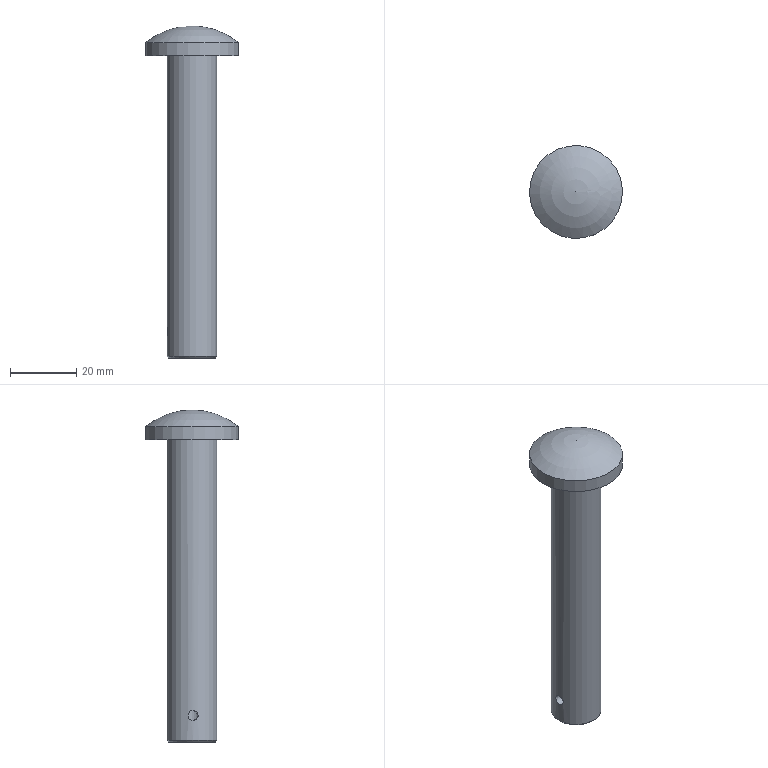Component | NX | RAM | 1 solid | 9 faces | volume 19578 mm3 | cylinder 4 | plane 2 | cone 2 | sphere 1 | commonest cylinder face diameters 15 x1 6 x1 28 x1 3 x1